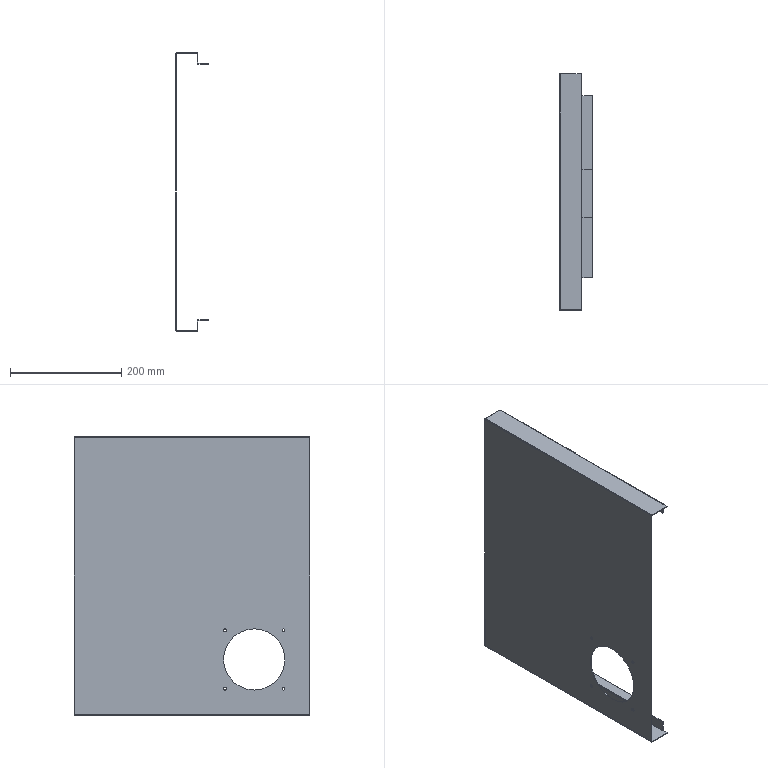Component | SolidWorks | WeldmentDrawing-1_LeftSidePanel-1 | 1 solid | 82 faces | volume 312837 mm3 | plane 59 | cylinder 23 | commonest cylinder face diameters 5 x8 0.2 x7 2.6 x6 110 x2